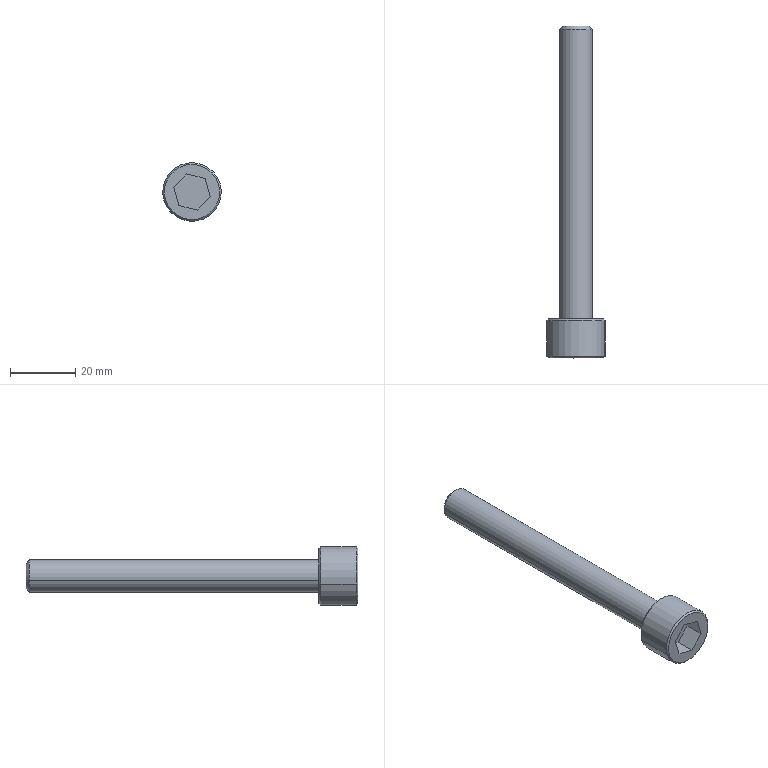Component | SolidWorks | 20-5 | 1 solid | 20 faces | box 18 x 102 x 18 mm | volume 9574 mm3 | plane 10 | cone 6 | cylinder 4 | commonest cylinder face diameters 10 x2 18 x2
STEP:
#1=COLOUR_RGB('',0.7922,0.8196,0.9333);
#2=FILL_AREA_STYLE_COLOUR('',#1);
#3=FILL_AREA_STYLE('',(#2));
#4=SURFACE_STYLE_FILL_AREA(#3);
#5=SURFACE_SIDE_STYLE('',(#4));
#6=SURFACE_STYLE_USAGE(.BOTH.,#5);
#7=PRESENTATION_STYLE_ASSIGNMENT((#6));
#8=CARTESIAN_POINT('',(1.857,-1.638,1.627));
#9=VERTEX_POINT('',#8);
#10=CARTESIAN_POINT('',(1.214,-1.638,1.444));
#11=VERTEX_POINT('',#10);
#12=CARTESIAN_POINT('',(1.535,-1.638,1.535));
#13=DIRECTION('',(0.,1.,-0.));
#14=DIRECTION('',(0.9619,0.,0.2733));
#15=AXIS2_PLACEMENT_3D('',#12,#13,#14);
#16=CIRCLE('',#15,0.3346);
#17=EDGE_CURVE('',#9,#11,#16,.T.);
#18=ORIENTED_EDGE('',*,*,#17,.F.);
#19=CARTESIAN_POINT('',(1.876,-1.657,1.632));
#20=VERTEX_POINT('',#19);
#21=CARTESIAN_POINT('',(1.857,-1.638,1.627));
#22=DIRECTION('',(0.6802,-0.7071,0.1932));
#23=VECTOR('',#22,39.37);
#24=LINE('',#21,#23);
#25=EDGE_CURVE('',#9,#20,#24,.T.);
#26=ORIENTED_EDGE('',*,*,#25,.T.);
#27=CARTESIAN_POINT('',(1.195,-1.657,1.439));
#28=VERTEX_POINT('',#27);
#29=CARTESIAN_POINT('',(1.535,-1.657,1.535));
#30=DIRECTION('',(-0.,-1.,0.));
#31=DIRECTION('',(0.9619,0.,0.2733));
#32=AXIS2_PLACEMENT_3D('',#29,#30,#31);
#33=CIRCLE('',#32,0.3543);
#34=EDGE_CURVE('',#28,#20,#33,.T.);
#35=ORIENTED_EDGE('',*,*,#34,.F.);
#36=CARTESIAN_POINT('',(1.214,-1.638,1.444));
#37=DIRECTION('',(-0.6802,-0.7071,-0.1932));
#38=VECTOR('',#37,39.37);
#39=LINE('',#36,#38);
#40=EDGE_CURVE('',#11,#28,#39,.T.);
#41=ORIENTED_EDGE('',*,*,#40,.F.);
#42=EDGE_LOOP('',(#18,#26,#35,#41));
#43=FACE_OUTER_BOUND('',#42,.T.);
#44=CARTESIAN_POINT('',(1.535,-1.638,1.535));
#45=DIRECTION('',(-0.,-1.,0.));
#46=DIRECTION('',(-0.9619,0.,-0.2733));
#47=AXIS2_PLACEMENT_3D('',#44,#45,#46);
#48=CONICAL_SURFACE('',#47,0.3346,0.7854);
#49=ADVANCED_FACE('',(#43),#48,.T.);
#50=CARTESIAN_POINT('',(1.214,-2.11,1.444));
#51=VERTEX_POINT('',#50);
#52=CARTESIAN_POINT('',(1.857,-2.11,1.627));
#53=VERTEX_POINT('',#52);
#54=CARTESIAN_POINT('',(1.535,-2.11,1.535));
#55=DIRECTION('',(-0.,-1.,0.));
#56=DIRECTION('',(0.9619,0.,0.2733));
#57=AXIS2_PLACEMENT_3D('',#54,#55,#56);
#58=CIRCLE('',#57,0.3346);
#59=EDGE_CURVE('',#51,#53,#58,.T.);
#60=ORIENTED_EDGE('',*,*,#59,.F.);
#61=CARTESIAN_POINT('',(1.195,-2.09,1.439));
#62=VERTEX_POINT('',#61);
#63=CARTESIAN_POINT('',(1.195,-2.09,1.439));
#64=DIRECTION('',(-0.6802,0.7071,-0.1932));
#65=VECTOR('',#64,39.37);
#66=LINE('',#63,#65);
#67=EDGE_CURVE('',#51,#62,#66,.T.);
#68=ORIENTED_EDGE('',*,*,#67,.T.);
#69=CARTESIAN_POINT('',(1.876,-2.09,1.632));
#70=VERTEX_POINT('',#69);
#71=CARTESIAN_POINT('',(1.535,-2.09,1.535));
#72=DIRECTION('',(0.,1.,-0.));
#73=DIRECTION('',(0.9619,0.,0.2733));
#74=AXIS2_PLACEMENT_3D('',#71,#72,#73);
#75=CIRCLE('',#74,0.3543);
#76=EDGE_CURVE('',#70,#62,#75,.T.);
#77=ORIENTED_EDGE('',*,*,#76,.F.);
#78=CARTESIAN_POINT('',(1.876,-2.09,1.632));
#79=DIRECTION('',(0.6802,0.7071,0.1932));
#80=VECTOR('',#79,39.37);
#81=LINE('',#78,#80);
#82=EDGE_CURVE('',#53,#70,#81,.T.);
#83=ORIENTED_EDGE('',*,*,#82,.F.);
#84=EDGE_LOOP('',(#60,#68,#77,#83));
#85=FACE_OUTER_BOUND('',#84,.T.);
#86=CARTESIAN_POINT('',(1.535,-2.09,1.535));
#87=DIRECTION('',(0.,1.,-0.));
#88=DIRECTION('',(0.9619,0.,0.2733));
#89=AXIS2_PLACEMENT_3D('',#86,#87,#88);
#90=CONICAL_SURFACE('',#89,0.3543,0.7854);
#91=ADVANCED_FACE('',(#85),#90,.T.);
#92=CARTESIAN_POINT('',(1.687,1.906,1.578));
#93=VERTEX_POINT('',#92);
#94=CARTESIAN_POINT('',(1.384,1.906,1.492));
#95=VERTEX_POINT('',#94);
#96=CARTESIAN_POINT('',(1.535,1.906,1.535));
#97=DIRECTION('',(0.,1.,-0.));
#98=DIRECTION('',(0.9619,0.,0.2733));
#99=AXIS2_PLACEMENT_3D('',#96,#97,#98);
#100=CIRCLE('',#99,0.1575);
#101=EDGE_CURVE('',#93,#95,#100,.T.);
#102=ORIENTED_EDGE('',*,*,#101,.F.);
#103=CARTESIAN_POINT('',(1.725,1.866,1.589));
#104=VERTEX_POINT('',#103);
#105=CARTESIAN_POINT('',(1.687,1.906,1.578));
#106=DIRECTION('',(0.6802,-0.7071,0.1932));
#107=VECTOR('',#106,39.37);
#108=LINE('',#105,#107);
#109=EDGE_CURVE('',#93,#104,#108,.T.);
#110=ORIENTED_EDGE('',*,*,#109,.T.);
#111=CARTESIAN_POINT('',(1.346,1.866,1.482));
#112=VERTEX_POINT('',#111);
#113=CARTESIAN_POINT('',(1.535,1.866,1.535));
#114=DIRECTION('',(-0.,-1.,0.));
#115=DIRECTION('',(0.9619,0.,0.2733));
#116=AXIS2_PLACEMENT_3D('',#113,#114,#115);
#117=CIRCLE('',#116,0.1969);
#118=EDGE_CURVE('',#112,#104,#117,.T.);
#119=ORIENTED_EDGE('',*,*,#118,.F.);
#120=CARTESIAN_POINT('',(1.384,1.906,1.492));
#121=DIRECTION('',(-0.6802,-0.7071,-0.1932));
#122=VECTOR('',#121,39.37);
#123=LINE('',#120,#122);
#124=EDGE_CURVE('',#95,#112,#123,.T.);
#125=ORIENTED_EDGE('',*,*,#124,.F.);
#126=EDGE_LOOP('',(#102,#110,#119,#125));
#127=FACE_OUTER_BOUND('',#126,.T.);
#128=CARTESIAN_POINT('',(1.535,1.906,1.535));
#129=DIRECTION('',(-0.,-1.,0.));
#130=DIRECTION('',(-0.9619,0.,-0.2733));
#131=AXIS2_PLACEMENT_3D('',#128,#129,#130);
#132=CONICAL_SURFACE('',#131,0.1575,0.7854);
#133=ADVANCED_FACE('',(#127),#132,.T.);
#134=ORIENTED_EDGE('',*,*,#118,.T.);
#135=CARTESIAN_POINT('',(1.725,-1.638,1.589));
#136=VERTEX_POINT('',#135);
#137=CARTESIAN_POINT('',(1.725,1.906,1.589));
#138=DIRECTION('',(-0.,-1.,0.));
#139=VECTOR('',#138,39.37);
#140=LINE('',#137,#139);
#141=EDGE_CURVE('',#104,#136,#140,.T.);
#142=ORIENTED_EDGE('',*,*,#141,.T.);
#143=CARTESIAN_POINT('',(1.346,-1.638,1.482));
#144=VERTEX_POINT('',#143);
#145=CARTESIAN_POINT('',(1.535,-1.638,1.535));
#146=DIRECTION('',(0.,1.,-0.));
#147=DIRECTION('',(0.9619,0.,0.2733));
#148=AXIS2_PLACEMENT_3D('',#145,#146,#147);
#149=CIRCLE('',#148,0.1969);
#150=EDGE_CURVE('',#136,#144,#149,.T.);
#151=ORIENTED_EDGE('',*,*,#150,.T.);
#152=CARTESIAN_POINT('',(1.346,1.906,1.482));
#153=DIRECTION('',(-0.,-1.,0.));
#154=VECTOR('',#153,39.37);
#155=LINE('',#152,#154);
#156=EDGE_CURVE('',#112,#144,#155,.T.);
#157=ORIENTED_EDGE('',*,*,#156,.F.);
#158=EDGE_LOOP('',(#134,#142,#151,#157));
#159=FACE_OUTER_BOUND('',#158,.T.);
#160=CARTESIAN_POINT('',(1.535,1.906,1.535));
#161=DIRECTION('',(-0.,-1.,0.));
#162=DIRECTION('',(-0.9619,0.,-0.2733));
#163=AXIS2_PLACEMENT_3D('',#160,#161,#162);
#164=CYLINDRICAL_SURFACE('',#163,0.1969);
#165=ADVANCED_FACE('',(#159),#164,.T.);
#166=ORIENTED_EDGE('',*,*,#34,.T.);
#167=CARTESIAN_POINT('',(1.876,-1.638,1.632));
#168=DIRECTION('',(-0.,-1.,0.));
#169=VECTOR('',#168,39.37);
#170=LINE('',#167,#169);
#171=EDGE_CURVE('',#20,#70,#170,.T.);
#172=ORIENTED_EDGE('',*,*,#171,.T.);
#173=ORIENTED_EDGE('',*,*,#76,.T.);
#174=CARTESIAN_POINT('',(1.195,-1.638,1.439));
#175=DIRECTION('',(-0.,-1.,0.));
#176=VECTOR('',#175,39.37);
#177=LINE('',#174,#176);
#178=EDGE_CURVE('',#28,#62,#177,.T.);
#179=ORIENTED_EDGE('',*,*,#178,.F.);
#180=EDGE_LOOP('',(#166,#172,#173,#179));
#181=FACE_OUTER_BOUND('',#180,.T.);
#182=CARTESIAN_POINT('',(1.535,-1.638,1.535));
#183=DIRECTION('',(-0.,-1.,0.));
#184=DIRECTION('',(-0.9619,0.,-0.2733));
#185=AXIS2_PLACEMENT_3D('',#182,#183,#184);
#186=CYLINDRICAL_SURFACE('',#185,0.3543);
#187=ADVANCED_FACE('',(#181),#186,.T.);
#188=ORIENTED_EDGE('',*,*,#171,.F.);
#189=CARTESIAN_POINT('',(1.535,-1.657,1.535));
#190=DIRECTION('',(-0.,-1.,0.));
#191=DIRECTION('',(0.9619,0.,0.2733));
#192=AXIS2_PLACEMENT_3D('',#189,#190,#191);
#193=CIRCLE('',#192,0.3543);
#194=EDGE_CURVE('',#20,#28,#193,.T.);
#195=ORIENTED_EDGE('',*,*,#194,.T.);
#196=ORIENTED_EDGE('',*,*,#178,.T.);
#197=CARTESIAN_POINT('',(1.535,-2.09,1.535));
#198=DIRECTION('',(0.,1.,-0.));
#199=DIRECTION('',(0.9619,0.,0.2733));
#200=AXIS2_PLACEMENT_3D('',#197,#198,#199);
#201=CIRCLE('',#200,0.3543);
#202=EDGE_CURVE('',#62,#70,#201,.T.);
#203=ORIENTED_EDGE('',*,*,#202,.T.);
#204=EDGE_LOOP('',(#188,#195,#196,#203));
#205=FACE_OUTER_BOUND('',#204,.T.);
#206=CARTESIAN_POINT('',(1.535,-1.638,1.535));
#207=DIRECTION('',(-0.,-1.,0.));
#208=DIRECTION('',(-0.9619,0.,-0.2733));
#209=AXIS2_PLACEMENT_3D('',#206,#207,#208);
#210=CYLINDRICAL_SURFACE('',#209,0.3543);
#211=ADVANCED_FACE('',(#205),#210,.T.);
#212=CARTESIAN_POINT('',(1.535,-1.638,1.535));
#213=DIRECTION('',(0.,1.,-0.));
#214=DIRECTION('',(0.9619,0.,0.2733));
#215=AXIS2_PLACEMENT_3D('',#212,#213,#214);
#216=CIRCLE('',#215,0.3346);
#217=EDGE_CURVE('',#11,#9,#216,.T.);
#218=ORIENTED_EDGE('',*,*,#217,.T.);
#219=ORIENTED_EDGE('',*,*,#17,.T.);
#220=EDGE_LOOP('',(#218,#219));
#221=FACE_OUTER_BOUND('',#220,.T.);
#222=CARTESIAN_POINT('',(1.535,-1.638,1.535));
#223=DIRECTION('',(0.,1.,-0.));
#224=DIRECTION('',(0.9619,0.,0.2733));
#225=AXIS2_PLACEMENT_3D('',#222,#223,#224);
#226=CIRCLE('',#225,0.1969);
#227=EDGE_CURVE('',#144,#136,#226,.T.);
#228=ORIENTED_EDGE('',*,*,#227,.F.);
#229=ORIENTED_EDGE('',*,*,#150,.F.);
#230=EDGE_LOOP('',(#228,#229));
#231=FACE_BOUND('',#230,.T.);
#232=CARTESIAN_POINT('',(1.535,-1.638,1.535));
#233=DIRECTION('',(0.,1.,-0.));
#234=DIRECTION('',(0.9619,-0.,0.2733));
#235=AXIS2_PLACEMENT_3D('',#232,#233,#234);
#236=PLANE('',#235);
#237=ADVANCED_FACE('',(#221,#231),#236,.T.);
#238=CARTESIAN_POINT('',(1.535,-2.11,1.535));
#239=DIRECTION('',(-0.,-1.,0.));
#240=DIRECTION('',(0.9619,0.,0.2733));
#241=AXIS2_PLACEMENT_3D('',#238,#239,#240);
#242=CIRCLE('',#241,0.3346);
#243=EDGE_CURVE('',#53,#51,#242,.T.);
#244=ORIENTED_EDGE('',*,*,#243,.T.);
#245=ORIENTED_EDGE('',*,*,#59,.T.);
#246=EDGE_LOOP('',(#244,#245));
#247=FACE_OUTER_BOUND('',#246,.T.);
#248=CARTESIAN_POINT('',(1.315,-2.11,1.591));
#249=VERTEX_POINT('',#248);
#250=CARTESIAN_POINT('',(1.377,-2.11,1.372));
#251=VERTEX_POINT('',#250);
#252=CARTESIAN_POINT('',(1.315,-2.11,1.591));
#253=DIRECTION('',(0.2733,-0.,-0.9619));
#254=VECTOR('',#253,39.37);
#255=LINE('',#252,#254);
#256=EDGE_CURVE('',#249,#251,#255,.T.);
#257=ORIENTED_EDGE('',*,*,#256,.F.);
#258=CARTESIAN_POINT('',(1.473,-2.11,1.754));
#259=VERTEX_POINT('',#258);
#260=CARTESIAN_POINT('',(1.473,-2.11,1.754));
#261=DIRECTION('',(-0.6964,-0.,-0.7176));
#262=VECTOR('',#261,39.37);
#263=LINE('',#260,#262);
#264=EDGE_CURVE('',#259,#249,#263,.T.);
#265=ORIENTED_EDGE('',*,*,#264,.F.);
#266=CARTESIAN_POINT('',(1.694,-2.11,1.699));
#267=VERTEX_POINT('',#266);
#268=CARTESIAN_POINT('',(1.694,-2.11,1.699));
#269=DIRECTION('',(-0.9697,0.,0.2443));
#270=VECTOR('',#269,39.37);
#271=LINE('',#268,#270);
#272=EDGE_CURVE('',#267,#259,#271,.T.);
#273=ORIENTED_EDGE('',*,*,#272,.F.);
#274=CARTESIAN_POINT('',(1.756,-2.11,1.48));
#275=VERTEX_POINT('',#274);
#276=CARTESIAN_POINT('',(1.756,-2.11,1.48));
#277=DIRECTION('',(-0.2733,0.,0.9619));
#278=VECTOR('',#277,39.37);
#279=LINE('',#276,#278);
#280=EDGE_CURVE('',#275,#267,#279,.T.);
#281=ORIENTED_EDGE('',*,*,#280,.F.);
#282=CARTESIAN_POINT('',(1.598,-2.11,1.317));
#283=VERTEX_POINT('',#282);
#284=CARTESIAN_POINT('',(1.598,-2.11,1.317));
#285=DIRECTION('',(0.6964,0.,0.7176));
#286=VECTOR('',#285,39.37);
#287=LINE('',#284,#286);
#288=EDGE_CURVE('',#283,#275,#287,.T.);
#289=ORIENTED_EDGE('',*,*,#288,.F.);
#290=CARTESIAN_POINT('',(1.377,-2.11,1.372));
#291=DIRECTION('',(0.9697,-0.,-0.2443));
#292=VECTOR('',#291,39.37);
#293=LINE('',#290,#292);
#294=EDGE_CURVE('',#251,#283,#293,.T.);
#295=ORIENTED_EDGE('',*,*,#294,.F.);
#296=EDGE_LOOP('',(#257,#265,#273,#281,#289,#295));
#297=FACE_BOUND('',#296,.T.);
#298=CARTESIAN_POINT('',(1.535,-2.11,1.535));
#299=DIRECTION('',(0.,1.,-0.));
#300=DIRECTION('',(0.9619,-0.,0.2733));
#301=AXIS2_PLACEMENT_3D('',#298,#299,#300);
#302=PLANE('',#301);
#303=ADVANCED_FACE('',(#247,#297),#302,.F.);
#304=ORIENTED_EDGE('',*,*,#141,.F.);
#305=CARTESIAN_POINT('',(1.535,1.866,1.535));
#306=DIRECTION('',(-0.,-1.,0.));
#307=DIRECTION('',(0.9619,0.,0.2733));
#308=AXIS2_PLACEMENT_3D('',#305,#306,#307);
#309=CIRCLE('',#308,0.1969);
#310=EDGE_CURVE('',#104,#112,#309,.T.);
#311=ORIENTED_EDGE('',*,*,#310,.T.);
#312=ORIENTED_EDGE('',*,*,#156,.T.);
#313=ORIENTED_EDGE('',*,*,#227,.T.);
#314=EDGE_LOOP('',(#304,#311,#312,#313));
#315=FACE_OUTER_BOUND('',#314,.T.);
#316=CARTESIAN_POINT('',(1.535,1.906,1.535));
#317=DIRECTION('',(-0.,-1.,0.));
#318=DIRECTION('',(-0.9619,0.,-0.2733));
#319=AXIS2_PLACEMENT_3D('',#316,#317,#318);
#320=CYLINDRICAL_SURFACE('',#319,0.1969);
#321=ADVANCED_FACE('',(#315),#320,.T.);
#322=CARTESIAN_POINT('',(1.535,1.906,1.535));
#323=DIRECTION('',(0.,1.,-0.));
#324=DIRECTION('',(0.9619,0.,0.2733));
#325=AXIS2_PLACEMENT_3D('',#322,#323,#324);
#326=CIRCLE('',#325,0.1575);
#327=EDGE_CURVE('',#95,#93,#326,.T.);
#328=ORIENTED_EDGE('',*,*,#327,.T.);
#329=ORIENTED_EDGE('',*,*,#101,.T.);
#330=EDGE_LOOP('',(#328,#329));
#331=FACE_OUTER_BOUND('',#330,.T.);
#332=CARTESIAN_POINT('',(1.535,1.906,1.535));
#333=DIRECTION('',(0.,1.,-0.));
#334=DIRECTION('',(0.9619,-0.,0.2733));
#335=AXIS2_PLACEMENT_3D('',#332,#333,#334);
#336=PLANE('',#335);
#337=ADVANCED_FACE('',(#331),#336,.T.);
#338=ORIENTED_EDGE('',*,*,#264,.T.);
#339=CARTESIAN_POINT('',(1.315,-1.874,1.591));
#340=VERTEX_POINT('',#339);
#341=CARTESIAN_POINT('',(1.315,-1.874,1.591));
#342=DIRECTION('',(-0.,-1.,0.));
#343=VECTOR('',#342,39.37);
#344=LINE('',#341,#343);
#345=EDGE_CURVE('',#340,#249,#344,.T.);
#346=ORIENTED_EDGE('',*,*,#345,.F.);
#347=CARTESIAN_POINT('',(1.473,-1.874,1.754));
#348=VERTEX_POINT('',#347);
#349=CARTESIAN_POINT('',(1.473,-1.874,1.754));
#350=DIRECTION('',(-0.6964,-0.,-0.7176));
#351=VECTOR('',#350,39.37);
#352=LINE('',#349,#351);
#353=EDGE_CURVE('',#348,#340,#352,.T.);
#354=ORIENTED_EDGE('',*,*,#353,.F.);
#355=CARTESIAN_POINT('',(1.473,-1.874,1.754));
#356=DIRECTION('',(-0.,-1.,0.));
#357=VECTOR('',#356,39.37);
#358=LINE('',#355,#357);
#359=EDGE_CURVE('',#348,#259,#358,.T.);
#360=ORIENTED_EDGE('',*,*,#359,.T.);
#361=EDGE_LOOP('',(#338,#346,#354,#360));
#362=FACE_OUTER_BOUND('',#361,.T.);
#363=CARTESIAN_POINT('',(1.473,-1.874,1.754));
#364=DIRECTION('',(-0.7176,0.,0.6964));
#365=DIRECTION('',(0.6964,0.,0.7176));
#366=AXIS2_PLACEMENT_3D('',#363,#364,#365);
#367=PLANE('',#366);
#368=ADVANCED_FACE('',(#362),#367,.F.);
#369=ORIENTED_EDGE('',*,*,#272,.T.);
#370=ORIENTED_EDGE('',*,*,#359,.F.);
#371=CARTESIAN_POINT('',(1.694,-1.874,1.699));
#372=VERTEX_POINT('',#371);
#373=CARTESIAN_POINT('',(1.694,-1.874,1.699));
#374=DIRECTION('',(-0.9697,0.,0.2443));
#375=VECTOR('',#374,39.37);
#376=LINE('',#373,#375);
#377=EDGE_CURVE('',#372,#348,#376,.T.);
#378=ORIENTED_EDGE('',*,*,#377,.F.);
#379=CARTESIAN_POINT('',(1.694,-1.874,1.699));
#380=DIRECTION('',(-0.,-1.,0.));
#381=VECTOR('',#380,39.37);
#382=LINE('',#379,#381);
#383=EDGE_CURVE('',#372,#267,#382,.T.);
#384=ORIENTED_EDGE('',*,*,#383,.T.);
#385=EDGE_LOOP('',(#369,#370,#378,#384));
#386=FACE_OUTER_BOUND('',#385,.T.);
#387=CARTESIAN_POINT('',(1.694,-1.874,1.699));
#388=DIRECTION('',(0.2443,0.,0.9697));
#389=DIRECTION('',(0.9697,-0.,-0.2443));
#390=AXIS2_PLACEMENT_3D('',#387,#388,#389);
#391=PLANE('',#390);
#392=ADVANCED_FACE('',(#386),#391,.F.);
#393=ORIENTED_EDGE('',*,*,#280,.T.);
#394=ORIENTED_EDGE('',*,*,#383,.F.);
#395=CARTESIAN_POINT('',(1.756,-1.874,1.48));
#396=VERTEX_POINT('',#395);
#397=CARTESIAN_POINT('',(1.756,-1.874,1.48));
#398=DIRECTION('',(-0.2733,0.,0.9619));
#399=VECTOR('',#398,39.37);
#400=LINE('',#397,#399);
#401=EDGE_CURVE('',#396,#372,#400,.T.);
#402=ORIENTED_EDGE('',*,*,#401,.F.);
#403=CARTESIAN_POINT('',(1.756,-1.874,1.48));
#404=DIRECTION('',(-0.,-1.,0.));
#405=VECTOR('',#404,39.37);
#406=LINE('',#403,#405);
#407=EDGE_CURVE('',#396,#275,#406,.T.);
#408=ORIENTED_EDGE('',*,*,#407,.T.);
#409=EDGE_LOOP('',(#393,#394,#402,#408));
#410=FACE_OUTER_BOUND('',#409,.T.);
#411=CARTESIAN_POINT('',(1.756,-1.874,1.48));
#412=DIRECTION('',(0.9619,-0.,0.2733));
#413=DIRECTION('',(0.2733,-0.,-0.9619));
#414=AXIS2_PLACEMENT_3D('',#411,#412,#413);
#415=PLANE('',#414);
#416=ADVANCED_FACE('',(#410),#415,.F.);
#417=ORIENTED_EDGE('',*,*,#288,.T.);
#418=ORIENTED_EDGE('',*,*,#407,.F.);
#419=CARTESIAN_POINT('',(1.598,-1.874,1.317));
#420=VERTEX_POINT('',#419);
#421=CARTESIAN_POINT('',(1.598,-1.874,1.317));
#422=DIRECTION('',(0.6964,0.,0.7176));
#423=VECTOR('',#422,39.37);
#424=LINE('',#421,#423);
#425=EDGE_CURVE('',#420,#396,#424,.T.);
#426=ORIENTED_EDGE('',*,*,#425,.F.);
#427=CARTESIAN_POINT('',(1.598,-1.874,1.317));
#428=DIRECTION('',(-0.,-1.,0.));
#429=VECTOR('',#428,39.37);
#430=LINE('',#427,#429);
#431=EDGE_CURVE('',#420,#283,#430,.T.);
#432=ORIENTED_EDGE('',*,*,#431,.T.);
#433=EDGE_LOOP('',(#417,#418,#426,#432));
#434=FACE_OUTER_BOUND('',#433,.T.);
#435=CARTESIAN_POINT('',(1.598,-1.874,1.317));
#436=DIRECTION('',(0.7176,-0.,-0.6964));
#437=DIRECTION('',(-0.6964,-0.,-0.7176));
#438=AXIS2_PLACEMENT_3D('',#435,#436,#437);
#439=PLANE('',#438);
#440=ADVANCED_FACE('',(#434),#439,.F.);
#441=ORIENTED_EDGE('',*,*,#294,.T.);
#442=ORIENTED_EDGE('',*,*,#431,.F.);
#443=CARTESIAN_POINT('',(1.377,-1.874,1.372));
#444=VERTEX_POINT('',#443);
#445=CARTESIAN_POINT('',(1.377,-1.874,1.372));
#446=DIRECTION('',(0.9697,-0.,-0.2443));
#447=VECTOR('',#446,39.37);
#448=LINE('',#445,#447);
#449=EDGE_CURVE('',#444,#420,#448,.T.);
#450=ORIENTED_EDGE('',*,*,#449,.F.);
#451=CARTESIAN_POINT('',(1.377,-1.874,1.372));
#452=DIRECTION('',(-0.,-1.,0.));
#453=VECTOR('',#452,39.37);
#454=LINE('',#451,#453);
#455=EDGE_CURVE('',#444,#251,#454,.T.);
#456=ORIENTED_EDGE('',*,*,#455,.T.);
#457=EDGE_LOOP('',(#441,#442,#450,#456));
#458=FACE_OUTER_BOUND('',#457,.T.);
#459=CARTESIAN_POINT('',(1.377,-1.874,1.372));
#460=DIRECTION('',(-0.2443,-0.,-0.9697));
#461=DIRECTION('',(-0.9697,0.,0.2443));
#462=AXIS2_PLACEMENT_3D('',#459,#460,#461);
#463=PLANE('',#462);
#464=ADVANCED_FACE('',(#458),#463,.F.);
#465=ORIENTED_EDGE('',*,*,#256,.T.);
#466=ORIENTED_EDGE('',*,*,#455,.F.);
#467=CARTESIAN_POINT('',(1.315,-1.874,1.591));
#468=DIRECTION('',(0.2733,-0.,-0.9619));
#469=VECTOR('',#468,39.37);
#470=LINE('',#467,#469);
#471=EDGE_CURVE('',#340,#444,#470,.T.);
#472=ORIENTED_EDGE('',*,*,#471,.F.);
#473=ORIENTED_EDGE('',*,*,#345,.T.);
#474=EDGE_LOOP('',(#465,#466,#472,#473));
#475=FACE_OUTER_BOUND('',#474,.T.);
#476=CARTESIAN_POINT('',(1.315,-1.874,1.591));
#477=DIRECTION('',(-0.9619,0.,-0.2733));
#478=DIRECTION('',(-0.2733,0.,0.9619));
#479=AXIS2_PLACEMENT_3D('',#476,#477,#478);
#480=PLANE('',#479);
#481=ADVANCED_FACE('',(#475),#480,.F.);
#482=ORIENTED_EDGE('',*,*,#353,.T.);
#483=ORIENTED_EDGE('',*,*,#471,.T.);
#484=ORIENTED_EDGE('',*,*,#449,.T.);
#485=ORIENTED_EDGE('',*,*,#425,.T.);
#486=ORIENTED_EDGE('',*,*,#401,.T.);
#487=ORIENTED_EDGE('',*,*,#377,.T.);
#488=EDGE_LOOP('',(#482,#483,#484,#485,#486,#487));
#489=FACE_OUTER_BOUND('',#488,.T.);
#490=CARTESIAN_POINT('',(1.535,-1.874,1.535));
#491=DIRECTION('',(-0.,-1.,0.));
#492=DIRECTION('',(-0.9619,0.,-0.2733));
#493=AXIS2_PLACEMENT_3D('',#490,#491,#492);
#494=PLANE('',#493);
#495=ADVANCED_FACE('',(#489),#494,.T.);
#496=ORIENTED_EDGE('',*,*,#109,.F.);
#497=ORIENTED_EDGE('',*,*,#327,.F.);
#498=ORIENTED_EDGE('',*,*,#124,.T.);
#499=ORIENTED_EDGE('',*,*,#310,.F.);
#500=EDGE_LOOP('',(#496,#497,#498,#499));
#501=FACE_OUTER_BOUND('',#500,.T.);
#502=CARTESIAN_POINT('',(1.535,1.906,1.535));
#503=DIRECTION('',(-0.,-1.,0.));
#504=DIRECTION('',(-0.9619,0.,-0.2733));
#505=AXIS2_PLACEMENT_3D('',#502,#503,#504);
#506=CONICAL_SURFACE('',#505,0.1575,0.7854);
#507=ADVANCED_FACE('',(#501),#506,.T.);
#508=ORIENTED_EDGE('',*,*,#67,.F.);
#509=ORIENTED_EDGE('',*,*,#243,.F.);
#510=ORIENTED_EDGE('',*,*,#82,.T.);
#511=ORIENTED_EDGE('',*,*,#202,.F.);
#512=EDGE_LOOP('',(#508,#509,#510,#511));
#513=FACE_OUTER_BOUND('',#512,.T.);
#514=CARTESIAN_POINT('',(1.535,-2.09,1.535));
#515=DIRECTION('',(0.,1.,-0.));
#516=DIRECTION('',(0.9619,0.,0.2733));
#517=AXIS2_PLACEMENT_3D('',#514,#515,#516);
#518=CONICAL_SURFACE('',#517,0.3543,0.7854);
#519=ADVANCED_FACE('',(#513),#518,.T.);
#520=ORIENTED_EDGE('',*,*,#25,.F.);
#521=ORIENTED_EDGE('',*,*,#217,.F.);
#522=ORIENTED_EDGE('',*,*,#40,.T.);
#523=ORIENTED_EDGE('',*,*,#194,.F.);
#524=EDGE_LOOP('',(#520,#521,#522,#523));
#525=FACE_OUTER_BOUND('',#524,.T.);
#526=CARTESIAN_POINT('',(1.535,-1.638,1.535));
#527=DIRECTION('',(-0.,-1.,0.));
#528=DIRECTION('',(-0.9619,0.,-0.2733));
#529=AXIS2_PLACEMENT_3D('',#526,#527,#528);
#530=CONICAL_SURFACE('',#529,0.3346,0.7854);
#531=ADVANCED_FACE('',(#525),#530,.T.);
#532=CLOSED_SHELL('',(#49,#91,#133,#165,#187,#211,#237,#303,#321,#337,#368,#392,#416,#440,#464,#481,#495,#507,#519,#531));
#533=MANIFOLD_SOLID_BREP('',#532);
#534=STYLED_ITEM('',(#7),#533);
#535=(LENGTH_UNIT()NAMED_UNIT(*)SI_UNIT($,.METRE.));
#536=LENGTH_MEASURE_WITH_UNIT(LENGTH_MEASURE(0.0254),#535);
#537=DIMENSIONAL_EXPONENTS(1.,0.,0.,0.,0.,0.,0.);
#538=(CONVERSION_BASED_UNIT('',#536)LENGTH_UNIT()NAMED_UNIT(#537));
#539=UNCERTAINTY_MEASURE_WITH_UNIT(LENGTH_MEASURE(0.00001),#538,'','');
#540=(NAMED_UNIT(*)PLANE_ANGLE_UNIT()SI_UNIT($,.RADIAN.));
#541=(NAMED_UNIT(*)SI_UNIT($,.STERADIAN.)SOLID_ANGLE_UNIT());
#542=(GEOMETRIC_REPRESENTATION_CONTEXT(3)GLOBAL_UNCERTAINTY_ASSIGNED_CONTEXT((#539))GLOBAL_UNIT_ASSIGNED_CONTEXT((#538,#540,#541))REPRESENTATION_CONTEXT('',''));
#543=MECHANICAL_DESIGN_GEOMETRIC_PRESENTATION_REPRESENTATION('',(#534),#542);
#544=CARTESIAN_POINT('',(0.,0.,0.));
#545=DIRECTION('',(0.,0.,1.));
#546=DIRECTION('',(1.,0.,0.));
#547=AXIS2_PLACEMENT_3D('',#544,#545,#546);
#548=(LENGTH_UNIT()NAMED_UNIT(*)SI_UNIT($,.METRE.));
#549=LENGTH_MEASURE_WITH_UNIT(LENGTH_MEASURE(0.0254),#548);
#550=DIMENSIONAL_EXPONENTS(1.,0.,0.,0.,0.,0.,0.);
#551=(CONVERSION_BASED_UNIT('',#549)LENGTH_UNIT()NAMED_UNIT(#550));
#552=UNCERTAINTY_MEASURE_WITH_UNIT(LENGTH_MEASURE(0.00001),#551,'','');
#553=(NAMED_UNIT(*)PLANE_ANGLE_UNIT()SI_UNIT($,.RADIAN.));
#554=(NAMED_UNIT(*)SI_UNIT($,.STERADIAN.)SOLID_ANGLE_UNIT());
#555=(GEOMETRIC_REPRESENTATION_CONTEXT(3)GLOBAL_UNCERTAINTY_ASSIGNED_CONTEXT((#552))GLOBAL_UNIT_ASSIGNED_CONTEXT((#551,#553,#554))REPRESENTATION_CONTEXT('',''));
#556=ADVANCED_BREP_SHAPE_REPRESENTATION('',(#533,#547),#555);
#557=PRESENTATION_LAYER_ASSIGNMENT('','',(#534));